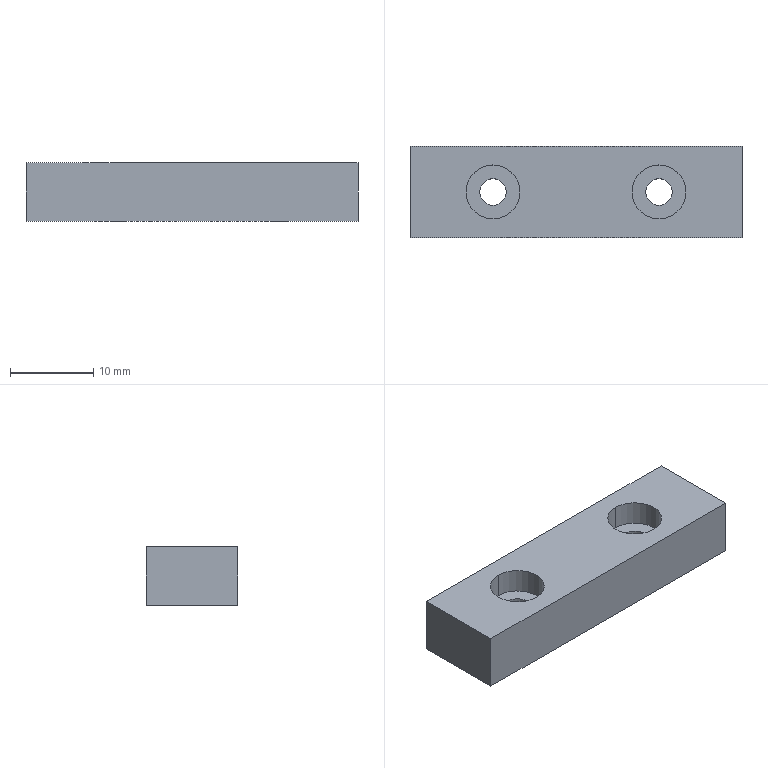Component | SolidWorks | SAWH02-03106A0MountingPlate6-8 | 1 solid | 16 faces | box 40 x 11 x 7 mm | volume 2817 mm3 | cylinder 8 | plane 8 | commonest cylinder face diameters 6.5 x4 3.2 x4 | material Polyurethane(Yellow)
build123d program:
from build123d import *

# Parameters (mm, degrees)
SKETCH1_W                                       = 40
SKETCH1_H                                       = 11
BOSS_EXTRUDE1_DEPTH                             = 7
M3_HEX_SOCKET_HEAD_CAP_SCREW_CBORE1_D           = 3.2
M3_HEX_SOCKET_HEAD_CAP_SCREW_CBORE1_CBORE_D     = 6.5
M3_HEX_SOCKET_HEAD_CAP_SCREW_CBORE1_CBORE_DEPTH = 3


with BuildPart() as part:
    # Sketch1 → Boss-Extrude1 (new body)
    with BuildSketch(Plane(origin=(0, 0, 0), x_dir=(1, 0, 0), z_dir=(0, 1, 0))):
        Rectangle(SKETCH1_W, SKETCH1_H)
    extrude(amount=BOSS_EXTRUDE1_DEPTH)

    # M3 Hex Socket Head Cap Screw CBORE1 (through all)
    with Locations(Plane(origin=(0, 7, 0), x_dir=(1, 0, 0), z_dir=(0, 1, 0))):
        with Locations((-10, 0), (10, 0)):
            CounterBoreHole(M3_HEX_SOCKET_HEAD_CAP_SCREW_CBORE1_D / 2, M3_HEX_SOCKET_HEAD_CAP_SCREW_CBORE1_CBORE_D / 2, M3_HEX_SOCKET_HEAD_CAP_SCREW_CBORE1_CBORE_DEPTH)


solid = part.part

# Placed as in the assembly
solid = solid.moved(Location((27.51, -6.388, -100.792), (90, 0, 0)))
STEP:
#1=COLOUR_RGB('',0.7922,0.8196,0.9333);
#2=FILL_AREA_STYLE_COLOUR('',#1);
#3=FILL_AREA_STYLE('',(#2));
#4=SURFACE_STYLE_FILL_AREA(#3);
#5=SURFACE_SIDE_STYLE('',(#4));
#6=SURFACE_STYLE_USAGE(.BOTH.,#5);
#7=PRESENTATION_STYLE_ASSIGNMENT((#6));
#8=CARTESIAN_POINT('',(0.6894,-0.1235,-3.811));
#9=VERTEX_POINT('',#8);
#10=CARTESIAN_POINT('',(0.6894,-0.3794,-3.811));
#11=VERTEX_POINT('',#10);
#12=CARTESIAN_POINT('',(0.6894,-0.2515,-3.811));
#13=DIRECTION('',(-0.,0.,1.));
#14=DIRECTION('',(0.,-1.,0.));
#15=AXIS2_PLACEMENT_3D('',#12,#13,#14);
#16=CIRCLE('',#15,0.128);
#17=EDGE_CURVE('',#9,#11,#16,.T.);
#18=ORIENTED_EDGE('',*,*,#17,.F.);
#19=CARTESIAN_POINT('',(0.6894,-0.1235,-3.693));
#20=VERTEX_POINT('',#19);
#21=CARTESIAN_POINT('',(0.6894,-0.1235,-3.693));
#22=DIRECTION('',(-0.,0.,1.));
#23=VECTOR('',#22,39.37);
#24=LINE('',#21,#23);
#25=EDGE_CURVE('',#9,#20,#24,.T.);
#26=ORIENTED_EDGE('',*,*,#25,.T.);
#27=CARTESIAN_POINT('',(0.6894,-0.3794,-3.693));
#28=VERTEX_POINT('',#27);
#29=CARTESIAN_POINT('',(0.6894,-0.2515,-3.693));
#30=DIRECTION('',(-0.,0.,1.));
#31=DIRECTION('',(0.,-1.,0.));
#32=AXIS2_PLACEMENT_3D('',#29,#30,#31);
#33=CIRCLE('',#32,0.128);
#34=EDGE_CURVE('',#20,#28,#33,.T.);
#35=ORIENTED_EDGE('',*,*,#34,.T.);
#36=CARTESIAN_POINT('',(0.6894,-0.3794,-3.693));
#37=DIRECTION('',(-0.,0.,1.));
#38=VECTOR('',#37,39.37);
#39=LINE('',#36,#38);
#40=EDGE_CURVE('',#11,#28,#39,.T.);
#41=ORIENTED_EDGE('',*,*,#40,.F.);
#42=EDGE_LOOP('',(#18,#26,#35,#41));
#43=FACE_OUTER_BOUND('',#42,.T.);
#44=CARTESIAN_POINT('',(0.6894,-0.2515,-3.693));
#45=DIRECTION('',(-0.,0.,1.));
#46=DIRECTION('',(0.,-1.,0.));
#47=AXIS2_PLACEMENT_3D('',#44,#45,#46);
#48=CYLINDRICAL_SURFACE('',#47,0.128);
#49=ADVANCED_FACE('',(#43),#48,.F.);
#50=CARTESIAN_POINT('',(0.6894,-0.1885,-3.968));
#51=VERTEX_POINT('',#50);
#52=CARTESIAN_POINT('',(0.6894,-0.3145,-3.968));
#53=VERTEX_POINT('',#52);
#54=CARTESIAN_POINT('',(0.6894,-0.2515,-3.968));
#55=DIRECTION('',(-0.,0.,1.));
#56=DIRECTION('',(0.,-1.,0.));
#57=AXIS2_PLACEMENT_3D('',#54,#55,#56);
#58=CIRCLE('',#57,0.06299);
#59=EDGE_CURVE('',#51,#53,#58,.T.);
#60=ORIENTED_EDGE('',*,*,#59,.F.);
#61=CARTESIAN_POINT('',(0.6894,-0.1885,-3.811));
#62=VERTEX_POINT('',#61);
#63=CARTESIAN_POINT('',(0.6894,-0.1885,-3.693));
#64=DIRECTION('',(-0.,0.,1.));
#65=VECTOR('',#64,39.37);
#66=LINE('',#63,#65);
#67=EDGE_CURVE('',#51,#62,#66,.T.);
#68=ORIENTED_EDGE('',*,*,#67,.T.);
#69=CARTESIAN_POINT('',(0.6894,-0.3145,-3.811));
#70=VERTEX_POINT('',#69);
#71=CARTESIAN_POINT('',(0.6894,-0.2515,-3.811));
#72=DIRECTION('',(-0.,0.,1.));
#73=DIRECTION('',(0.,-1.,0.));
#74=AXIS2_PLACEMENT_3D('',#71,#72,#73);
#75=CIRCLE('',#74,0.06299);
#76=EDGE_CURVE('',#62,#70,#75,.T.);
#77=ORIENTED_EDGE('',*,*,#76,.T.);
#78=CARTESIAN_POINT('',(0.6894,-0.3145,-3.693));
#79=DIRECTION('',(-0.,0.,1.));
#80=VECTOR('',#79,39.37);
#81=LINE('',#78,#80);
#82=EDGE_CURVE('',#53,#70,#81,.T.);
#83=ORIENTED_EDGE('',*,*,#82,.F.);
#84=EDGE_LOOP('',(#60,#68,#77,#83));
#85=FACE_OUTER_BOUND('',#84,.T.);
#86=CARTESIAN_POINT('',(0.6894,-0.2515,-3.693));
#87=DIRECTION('',(-0.,0.,1.));
#88=DIRECTION('',(0.,-1.,0.));
#89=AXIS2_PLACEMENT_3D('',#86,#87,#88);
#90=CYLINDRICAL_SURFACE('',#89,0.06299);
#91=ADVANCED_FACE('',(#85),#90,.F.);
#92=CARTESIAN_POINT('',(1.477,-0.1235,-3.811));
#93=VERTEX_POINT('',#92);
#94=CARTESIAN_POINT('',(1.477,-0.3794,-3.811));
#95=VERTEX_POINT('',#94);
#96=CARTESIAN_POINT('',(1.477,-0.2515,-3.811));
#97=DIRECTION('',(-0.,0.,1.));
#98=DIRECTION('',(0.,-1.,0.));
#99=AXIS2_PLACEMENT_3D('',#96,#97,#98);
#100=CIRCLE('',#99,0.128);
#101=EDGE_CURVE('',#93,#95,#100,.T.);
#102=ORIENTED_EDGE('',*,*,#101,.F.);
#103=CARTESIAN_POINT('',(1.477,-0.1235,-3.693));
#104=VERTEX_POINT('',#103);
#105=CARTESIAN_POINT('',(1.477,-0.1235,-3.693));
#106=DIRECTION('',(-0.,0.,1.));
#107=VECTOR('',#106,39.37);
#108=LINE('',#105,#107);
#109=EDGE_CURVE('',#93,#104,#108,.T.);
#110=ORIENTED_EDGE('',*,*,#109,.T.);
#111=CARTESIAN_POINT('',(1.477,-0.3794,-3.693));
#112=VERTEX_POINT('',#111);
#113=CARTESIAN_POINT('',(1.477,-0.2515,-3.693));
#114=DIRECTION('',(-0.,0.,1.));
#115=DIRECTION('',(0.,-1.,0.));
#116=AXIS2_PLACEMENT_3D('',#113,#114,#115);
#117=CIRCLE('',#116,0.128);
#118=EDGE_CURVE('',#104,#112,#117,.T.);
#119=ORIENTED_EDGE('',*,*,#118,.T.);
#120=CARTESIAN_POINT('',(1.477,-0.3794,-3.693));
#121=DIRECTION('',(-0.,0.,1.));
#122=VECTOR('',#121,39.37);
#123=LINE('',#120,#122);
#124=EDGE_CURVE('',#95,#112,#123,.T.);
#125=ORIENTED_EDGE('',*,*,#124,.F.);
#126=EDGE_LOOP('',(#102,#110,#119,#125));
#127=FACE_OUTER_BOUND('',#126,.T.);
#128=CARTESIAN_POINT('',(1.477,-0.2515,-3.693));
#129=DIRECTION('',(-0.,0.,1.));
#130=DIRECTION('',(0.,-1.,0.));
#131=AXIS2_PLACEMENT_3D('',#128,#129,#130);
#132=CYLINDRICAL_SURFACE('',#131,0.128);
#133=ADVANCED_FACE('',(#127),#132,.F.);
#134=CARTESIAN_POINT('',(1.477,-0.1885,-3.968));
#135=VERTEX_POINT('',#134);
#136=CARTESIAN_POINT('',(1.477,-0.3145,-3.968));
#137=VERTEX_POINT('',#136);
#138=CARTESIAN_POINT('',(1.477,-0.2515,-3.968));
#139=DIRECTION('',(-0.,0.,1.));
#140=DIRECTION('',(0.,-1.,0.));
#141=AXIS2_PLACEMENT_3D('',#138,#139,#140);
#142=CIRCLE('',#141,0.06299);
#143=EDGE_CURVE('',#135,#137,#142,.T.);
#144=ORIENTED_EDGE('',*,*,#143,.F.);
#145=CARTESIAN_POINT('',(1.477,-0.1885,-3.811));
#146=VERTEX_POINT('',#145);
#147=CARTESIAN_POINT('',(1.477,-0.1885,-3.693));
#148=DIRECTION('',(-0.,0.,1.));
#149=VECTOR('',#148,39.37);
#150=LINE('',#147,#149);
#151=EDGE_CURVE('',#135,#146,#150,.T.);
#152=ORIENTED_EDGE('',*,*,#151,.T.);
#153=CARTESIAN_POINT('',(1.477,-0.3145,-3.811));
#154=VERTEX_POINT('',#153);
#155=CARTESIAN_POINT('',(1.477,-0.2515,-3.811));
#156=DIRECTION('',(-0.,0.,1.));
#157=DIRECTION('',(0.,-1.,0.));
#158=AXIS2_PLACEMENT_3D('',#155,#156,#157);
#159=CIRCLE('',#158,0.06299);
#160=EDGE_CURVE('',#146,#154,#159,.T.);
#161=ORIENTED_EDGE('',*,*,#160,.T.);
#162=CARTESIAN_POINT('',(1.477,-0.3145,-3.693));
#163=DIRECTION('',(-0.,0.,1.));
#164=VECTOR('',#163,39.37);
#165=LINE('',#162,#164);
#166=EDGE_CURVE('',#137,#154,#165,.T.);
#167=ORIENTED_EDGE('',*,*,#166,.F.);
#168=EDGE_LOOP('',(#144,#152,#161,#167));
#169=FACE_OUTER_BOUND('',#168,.T.);
#170=CARTESIAN_POINT('',(1.477,-0.2515,-3.693));
#171=DIRECTION('',(-0.,0.,1.));
#172=DIRECTION('',(0.,-1.,0.));
#173=AXIS2_PLACEMENT_3D('',#170,#171,#172);
#174=CYLINDRICAL_SURFACE('',#173,0.06299);
#175=ADVANCED_FACE('',(#169),#174,.F.);
#176=CARTESIAN_POINT('',(0.2957,-0.03495,-3.968));
#177=VERTEX_POINT('',#176);
#178=CARTESIAN_POINT('',(0.2957,-0.468,-3.968));
#179=VERTEX_POINT('',#178);
#180=CARTESIAN_POINT('',(0.2957,-0.03495,-3.968));
#181=DIRECTION('',(-0.,-1.,0.));
#182=VECTOR('',#181,39.37);
#183=LINE('',#180,#182);
#184=EDGE_CURVE('',#177,#179,#183,.T.);
#185=ORIENTED_EDGE('',*,*,#184,.T.);
#186=CARTESIAN_POINT('',(0.2957,-0.468,-3.693));
#187=VERTEX_POINT('',#186);
#188=CARTESIAN_POINT('',(0.2957,-0.468,-3.693));
#189=DIRECTION('',(0.,-0.,-1.));
#190=VECTOR('',#189,39.37);
#191=LINE('',#188,#190);
#192=EDGE_CURVE('',#187,#179,#191,.T.);
#193=ORIENTED_EDGE('',*,*,#192,.F.);
#194=CARTESIAN_POINT('',(0.2957,-0.03495,-3.693));
#195=VERTEX_POINT('',#194);
#196=CARTESIAN_POINT('',(0.2957,-0.03495,-3.693));
#197=DIRECTION('',(-0.,-1.,0.));
#198=VECTOR('',#197,39.37);
#199=LINE('',#196,#198);
#200=EDGE_CURVE('',#195,#187,#199,.T.);
#201=ORIENTED_EDGE('',*,*,#200,.F.);
#202=CARTESIAN_POINT('',(0.2957,-0.03495,-3.693));
#203=DIRECTION('',(0.,-0.,-1.));
#204=VECTOR('',#203,39.37);
#205=LINE('',#202,#204);
#206=EDGE_CURVE('',#195,#177,#205,.T.);
#207=ORIENTED_EDGE('',*,*,#206,.T.);
#208=EDGE_LOOP('',(#185,#193,#201,#207));
#209=FACE_OUTER_BOUND('',#208,.T.);
#210=CARTESIAN_POINT('',(0.2957,-0.03495,-3.693));
#211=DIRECTION('',(1.,-0.,0.));
#212=DIRECTION('',(0.,1.,-0.));
#213=AXIS2_PLACEMENT_3D('',#210,#211,#212);
#214=PLANE('',#213);
#215=ADVANCED_FACE('',(#209),#214,.F.);
#216=CARTESIAN_POINT('',(1.87,-0.468,-3.968));
#217=VERTEX_POINT('',#216);
#218=CARTESIAN_POINT('',(0.2957,-0.468,-3.968));
#219=DIRECTION('',(1.,-0.,0.));
#220=VECTOR('',#219,39.37);
#221=LINE('',#218,#220);
#222=EDGE_CURVE('',#179,#217,#221,.T.);
#223=ORIENTED_EDGE('',*,*,#222,.T.);
#224=CARTESIAN_POINT('',(1.87,-0.468,-3.693));
#225=VERTEX_POINT('',#224);
#226=CARTESIAN_POINT('',(1.87,-0.468,-3.693));
#227=DIRECTION('',(0.,-0.,-1.));
#228=VECTOR('',#227,39.37);
#229=LINE('',#226,#228);
#230=EDGE_CURVE('',#225,#217,#229,.T.);
#231=ORIENTED_EDGE('',*,*,#230,.F.);
#232=CARTESIAN_POINT('',(0.2957,-0.468,-3.693));
#233=DIRECTION('',(1.,-0.,0.));
#234=VECTOR('',#233,39.37);
#235=LINE('',#232,#234);
#236=EDGE_CURVE('',#187,#225,#235,.T.);
#237=ORIENTED_EDGE('',*,*,#236,.F.);
#238=ORIENTED_EDGE('',*,*,#192,.T.);
#239=EDGE_LOOP('',(#223,#231,#237,#238));
#240=FACE_OUTER_BOUND('',#239,.T.);
#241=CARTESIAN_POINT('',(0.2957,-0.468,-3.693));
#242=DIRECTION('',(0.,1.,-0.));
#243=DIRECTION('',(-1.,0.,-0.));
#244=AXIS2_PLACEMENT_3D('',#241,#242,#243);
#245=PLANE('',#244);
#246=ADVANCED_FACE('',(#240),#245,.F.);
#247=CARTESIAN_POINT('',(1.87,-0.03495,-3.968));
#248=VERTEX_POINT('',#247);
#249=CARTESIAN_POINT('',(1.87,-0.03495,-3.968));
#250=DIRECTION('',(0.,1.,-0.));
#251=VECTOR('',#250,39.37);
#252=LINE('',#249,#251);
#253=EDGE_CURVE('',#217,#248,#252,.T.);
#254=ORIENTED_EDGE('',*,*,#253,.T.);
#255=CARTESIAN_POINT('',(1.87,-0.03495,-3.693));
#256=VERTEX_POINT('',#255);
#257=CARTESIAN_POINT('',(1.87,-0.03495,-3.693));
#258=DIRECTION('',(0.,-0.,-1.));
#259=VECTOR('',#258,39.37);
#260=LINE('',#257,#259);
#261=EDGE_CURVE('',#256,#248,#260,.T.);
#262=ORIENTED_EDGE('',*,*,#261,.F.);
#263=CARTESIAN_POINT('',(1.87,-0.03495,-3.693));
#264=DIRECTION('',(0.,1.,-0.));
#265=VECTOR('',#264,39.37);
#266=LINE('',#263,#265);
#267=EDGE_CURVE('',#225,#256,#266,.T.);
#268=ORIENTED_EDGE('',*,*,#267,.F.);
#269=ORIENTED_EDGE('',*,*,#230,.T.);
#270=EDGE_LOOP('',(#254,#262,#268,#269));
#271=FACE_OUTER_BOUND('',#270,.T.);
#272=CARTESIAN_POINT('',(1.87,-0.03495,-3.693));
#273=DIRECTION('',(-1.,0.,-0.));
#274=DIRECTION('',(-0.,-1.,0.));
#275=AXIS2_PLACEMENT_3D('',#272,#273,#274);
#276=PLANE('',#275);
#277=ADVANCED_FACE('',(#271),#276,.F.);
#278=CARTESIAN_POINT('',(0.2957,-0.03495,-3.968));
#279=DIRECTION('',(-1.,0.,-0.));
#280=VECTOR('',#279,39.37);
#281=LINE('',#278,#280);
#282=EDGE_CURVE('',#248,#177,#281,.T.);
#283=ORIENTED_EDGE('',*,*,#282,.T.);
#284=ORIENTED_EDGE('',*,*,#206,.F.);
#285=CARTESIAN_POINT('',(0.2957,-0.03495,-3.693));
#286=DIRECTION('',(-1.,0.,-0.));
#287=VECTOR('',#286,39.37);
#288=LINE('',#285,#287);
#289=EDGE_CURVE('',#256,#195,#288,.T.);
#290=ORIENTED_EDGE('',*,*,#289,.F.);
#291=ORIENTED_EDGE('',*,*,#261,.T.);
#292=EDGE_LOOP('',(#283,#284,#290,#291));
#293=FACE_OUTER_BOUND('',#292,.T.);
#294=CARTESIAN_POINT('',(0.2957,-0.03495,-3.693));
#295=DIRECTION('',(-0.,-1.,0.));
#296=DIRECTION('',(1.,-0.,0.));
#297=AXIS2_PLACEMENT_3D('',#294,#295,#296);
#298=PLANE('',#297);
#299=ADVANCED_FACE('',(#293),#298,.F.);
#300=CARTESIAN_POINT('',(0.6894,-0.2515,-3.693));
#301=DIRECTION('',(-0.,0.,1.));
#302=DIRECTION('',(0.,-1.,0.));
#303=AXIS2_PLACEMENT_3D('',#300,#301,#302);
#304=CIRCLE('',#303,0.128);
#305=EDGE_CURVE('',#28,#20,#304,.T.);
#306=ORIENTED_EDGE('',*,*,#305,.F.);
#307=ORIENTED_EDGE('',*,*,#34,.F.);
#308=EDGE_LOOP('',(#306,#307));
#309=FACE_BOUND('',#308,.T.);
#310=CARTESIAN_POINT('',(1.477,-0.2515,-3.693));
#311=DIRECTION('',(-0.,0.,1.));
#312=DIRECTION('',(0.,-1.,0.));
#313=AXIS2_PLACEMENT_3D('',#310,#311,#312);
#314=CIRCLE('',#313,0.128);
#315=EDGE_CURVE('',#112,#104,#314,.T.);
#316=ORIENTED_EDGE('',*,*,#315,.F.);
#317=ORIENTED_EDGE('',*,*,#118,.F.);
#318=EDGE_LOOP('',(#316,#317));
#319=FACE_BOUND('',#318,.T.);
#320=ORIENTED_EDGE('',*,*,#200,.T.);
#321=ORIENTED_EDGE('',*,*,#236,.T.);
#322=ORIENTED_EDGE('',*,*,#267,.T.);
#323=ORIENTED_EDGE('',*,*,#289,.T.);
#324=EDGE_LOOP('',(#320,#321,#322,#323));
#325=FACE_OUTER_BOUND('',#324,.T.);
#326=CARTESIAN_POINT('',(1.083,-0.2515,-3.693));
#327=DIRECTION('',(-0.,0.,1.));
#328=DIRECTION('',(-0.,-1.,0.));
#329=AXIS2_PLACEMENT_3D('',#326,#327,#328);
#330=PLANE('',#329);
#331=ADVANCED_FACE('',(#309,#319,#325),#330,.T.);
#332=CARTESIAN_POINT('',(0.6894,-0.2515,-3.968));
#333=DIRECTION('',(-0.,0.,1.));
#334=DIRECTION('',(0.,-1.,0.));
#335=AXIS2_PLACEMENT_3D('',#332,#333,#334);
#336=CIRCLE('',#335,0.06299);
#337=EDGE_CURVE('',#53,#51,#336,.T.);
#338=ORIENTED_EDGE('',*,*,#337,.T.);
#339=ORIENTED_EDGE('',*,*,#59,.T.);
#340=EDGE_LOOP('',(#338,#339));
#341=FACE_BOUND('',#340,.T.);
#342=CARTESIAN_POINT('',(1.477,-0.2515,-3.968));
#343=DIRECTION('',(-0.,0.,1.));
#344=DIRECTION('',(0.,-1.,0.));
#345=AXIS2_PLACEMENT_3D('',#342,#343,#344);
#346=CIRCLE('',#345,0.06299);
#347=EDGE_CURVE('',#137,#135,#346,.T.);
#348=ORIENTED_EDGE('',*,*,#347,.T.);
#349=ORIENTED_EDGE('',*,*,#143,.T.);
#350=EDGE_LOOP('',(#348,#349));
#351=FACE_BOUND('',#350,.T.);
#352=ORIENTED_EDGE('',*,*,#184,.F.);
#353=ORIENTED_EDGE('',*,*,#282,.F.);
#354=ORIENTED_EDGE('',*,*,#253,.F.);
#355=ORIENTED_EDGE('',*,*,#222,.F.);
#356=EDGE_LOOP('',(#352,#353,#354,#355));
#357=FACE_OUTER_BOUND('',#356,.T.);
#358=CARTESIAN_POINT('',(1.083,-0.2515,-3.968));
#359=DIRECTION('',(-0.,0.,1.));
#360=DIRECTION('',(-0.,-1.,0.));
#361=AXIS2_PLACEMENT_3D('',#358,#359,#360);
#362=PLANE('',#361);
#363=ADVANCED_FACE('',(#341,#351,#357),#362,.F.);
#364=ORIENTED_EDGE('',*,*,#151,.F.);
#365=ORIENTED_EDGE('',*,*,#347,.F.);
#366=ORIENTED_EDGE('',*,*,#166,.T.);
#367=CARTESIAN_POINT('',(1.477,-0.2515,-3.811));
#368=DIRECTION('',(-0.,0.,1.));
#369=DIRECTION('',(0.,-1.,0.));
#370=AXIS2_PLACEMENT_3D('',#367,#368,#369);
#371=CIRCLE('',#370,0.06299);
#372=EDGE_CURVE('',#154,#146,#371,.T.);
#373=ORIENTED_EDGE('',*,*,#372,.T.);
#374=EDGE_LOOP('',(#364,#365,#366,#373));
#375=FACE_OUTER_BOUND('',#374,.T.);
#376=CARTESIAN_POINT('',(1.477,-0.2515,-3.693));
#377=DIRECTION('',(-0.,0.,1.));
#378=DIRECTION('',(0.,-1.,0.));
#379=AXIS2_PLACEMENT_3D('',#376,#377,#378);
#380=CYLINDRICAL_SURFACE('',#379,0.06299);
#381=ADVANCED_FACE('',(#375),#380,.F.);
#382=ORIENTED_EDGE('',*,*,#372,.F.);
#383=ORIENTED_EDGE('',*,*,#160,.F.);
#384=EDGE_LOOP('',(#382,#383));
#385=FACE_BOUND('',#384,.T.);
#386=CARTESIAN_POINT('',(1.477,-0.2515,-3.811));
#387=DIRECTION('',(-0.,0.,1.));
#388=DIRECTION('',(0.,-1.,0.));
#389=AXIS2_PLACEMENT_3D('',#386,#387,#388);
#390=CIRCLE('',#389,0.128);
#391=EDGE_CURVE('',#95,#93,#390,.T.);
#392=ORIENTED_EDGE('',*,*,#391,.T.);
#393=ORIENTED_EDGE('',*,*,#101,.T.);
#394=EDGE_LOOP('',(#392,#393));
#395=FACE_OUTER_BOUND('',#394,.T.);
#396=CARTESIAN_POINT('',(1.54,-0.2515,-3.811));
#397=DIRECTION('',(0.,-0.,-1.));
#398=DIRECTION('',(0.,1.,-0.));
#399=AXIS2_PLACEMENT_3D('',#396,#397,#398);
#400=PLANE('',#399);
#401=ADVANCED_FACE('',(#385,#395),#400,.F.);
#402=ORIENTED_EDGE('',*,*,#109,.F.);
#403=ORIENTED_EDGE('',*,*,#391,.F.);
#404=ORIENTED_EDGE('',*,*,#124,.T.);
#405=ORIENTED_EDGE('',*,*,#315,.T.);
#406=EDGE_LOOP('',(#402,#403,#404,#405));
#407=FACE_OUTER_BOUND('',#406,.T.);
#408=CARTESIAN_POINT('',(1.477,-0.2515,-3.693));
#409=DIRECTION('',(-0.,0.,1.));
#410=DIRECTION('',(0.,-1.,0.));
#411=AXIS2_PLACEMENT_3D('',#408,#409,#410);
#412=CYLINDRICAL_SURFACE('',#411,0.128);
#413=ADVANCED_FACE('',(#407),#412,.F.);
#414=ORIENTED_EDGE('',*,*,#67,.F.);
#415=ORIENTED_EDGE('',*,*,#337,.F.);
#416=ORIENTED_EDGE('',*,*,#82,.T.);
#417=CARTESIAN_POINT('',(0.6894,-0.2515,-3.811));
#418=DIRECTION('',(-0.,0.,1.));
#419=DIRECTION('',(0.,-1.,0.));
#420=AXIS2_PLACEMENT_3D('',#417,#418,#419);
#421=CIRCLE('',#420,0.06299);
#422=EDGE_CURVE('',#70,#62,#421,.T.);
#423=ORIENTED_EDGE('',*,*,#422,.T.);
#424=EDGE_LOOP('',(#414,#415,#416,#423));
#425=FACE_OUTER_BOUND('',#424,.T.);
#426=CARTESIAN_POINT('',(0.6894,-0.2515,-3.693));
#427=DIRECTION('',(-0.,0.,1.));
#428=DIRECTION('',(0.,-1.,0.));
#429=AXIS2_PLACEMENT_3D('',#426,#427,#428);
#430=CYLINDRICAL_SURFACE('',#429,0.06299);
#431=ADVANCED_FACE('',(#425),#430,.F.);
#432=ORIENTED_EDGE('',*,*,#422,.F.);
#433=ORIENTED_EDGE('',*,*,#76,.F.);
#434=EDGE_LOOP('',(#432,#433));
#435=FACE_BOUND('',#434,.T.);
#436=CARTESIAN_POINT('',(0.6894,-0.2515,-3.811));
#437=DIRECTION('',(-0.,0.,1.));
#438=DIRECTION('',(0.,-1.,0.));
#439=AXIS2_PLACEMENT_3D('',#436,#437,#438);
#440=CIRCLE('',#439,0.128);
#441=EDGE_CURVE('',#11,#9,#440,.T.);
#442=ORIENTED_EDGE('',*,*,#441,.T.);
#443=ORIENTED_EDGE('',*,*,#17,.T.);
#444=EDGE_LOOP('',(#442,#443));
#445=FACE_OUTER_BOUND('',#444,.T.);
#446=CARTESIAN_POINT('',(0.7524,-0.2515,-3.811));
#447=DIRECTION('',(0.,-0.,-1.));
#448=DIRECTION('',(0.,1.,-0.));
#449=AXIS2_PLACEMENT_3D('',#446,#447,#448);
#450=PLANE('',#449);
#451=ADVANCED_FACE('',(#435,#445),#450,.F.);
#452=ORIENTED_EDGE('',*,*,#25,.F.);
#453=ORIENTED_EDGE('',*,*,#441,.F.);
#454=ORIENTED_EDGE('',*,*,#40,.T.);
#455=ORIENTED_EDGE('',*,*,#305,.T.);
#456=EDGE_LOOP('',(#452,#453,#454,#455));
#457=FACE_OUTER_BOUND('',#456,.T.);
#458=CARTESIAN_POINT('',(0.6894,-0.2515,-3.693));
#459=DIRECTION('',(-0.,0.,1.));
#460=DIRECTION('',(0.,-1.,0.));
#461=AXIS2_PLACEMENT_3D('',#458,#459,#460);
#462=CYLINDRICAL_SURFACE('',#461,0.128);
#463=ADVANCED_FACE('',(#457),#462,.F.);
#464=CLOSED_SHELL('',(#49,#91,#133,#175,#215,#246,#277,#299,#331,#363,#381,#401,#413,#431,#451,#463));
#465=MANIFOLD_SOLID_BREP('',#464);
#466=STYLED_ITEM('',(#7),#465);
#467=PRESENTATION_LAYER_ASSIGNMENT('','',(#466));
#468=CARTESIAN_POINT('',(0.,0.,0.));
#469=DIRECTION('',(0.,0.,1.));
#470=DIRECTION('',(1.,0.,0.));
#471=AXIS2_PLACEMENT_3D('',#468,#469,#470);
#472=(LENGTH_UNIT()NAMED_UNIT(*)SI_UNIT($,.METRE.));
#473=LENGTH_MEASURE_WITH_UNIT(LENGTH_MEASURE(0.0254),#472);
#474=DIMENSIONAL_EXPONENTS(1.,0.,0.,0.,0.,0.,0.);
#475=(CONVERSION_BASED_UNIT('',#473)LENGTH_UNIT()NAMED_UNIT(#474));
#476=UNCERTAINTY_MEASURE_WITH_UNIT(LENGTH_MEASURE(0.00001),#475,'','');
#477=(NAMED_UNIT(*)PLANE_ANGLE_UNIT()SI_UNIT($,.RADIAN.));
#478=(NAMED_UNIT(*)SI_UNIT($,.STERADIAN.)SOLID_ANGLE_UNIT());
#479=(GEOMETRIC_REPRESENTATION_CONTEXT(3)GLOBAL_UNCERTAINTY_ASSIGNED_CONTEXT((#476))GLOBAL_UNIT_ASSIGNED_CONTEXT((#475,#477,#478))REPRESENTATION_CONTEXT('',''));
#480=ADVANCED_BREP_SHAPE_REPRESENTATION('',(#465,#471),#479);
#481=(LENGTH_UNIT()NAMED_UNIT(*)SI_UNIT($,.METRE.));
#482=LENGTH_MEASURE_WITH_UNIT(LENGTH_MEASURE(0.0254),#481);
#483=DIMENSIONAL_EXPONENTS(1.,0.,0.,0.,0.,0.,0.);
#484=(CONVERSION_BASED_UNIT('',#482)LENGTH_UNIT()NAMED_UNIT(#483));
#485=UNCERTAINTY_MEASURE_WITH_UNIT(LENGTH_MEASURE(0.00001),#484,'','');
#486=(NAMED_UNIT(*)PLANE_ANGLE_UNIT()SI_UNIT($,.RADIAN.));
#487=(NAMED_UNIT(*)SI_UNIT($,.STERADIAN.)SOLID_ANGLE_UNIT());
#488=(GEOMETRIC_REPRESENTATION_CONTEXT(3)GLOBAL_UNCERTAINTY_ASSIGNED_CONTEXT((#485))GLOBAL_UNIT_ASSIGNED_CONTEXT((#484,#486,#487))REPRESENTATION_CONTEXT('',''));
#489=MECHANICAL_DESIGN_GEOMETRIC_PRESENTATION_REPRESENTATION('',(#466),#488);